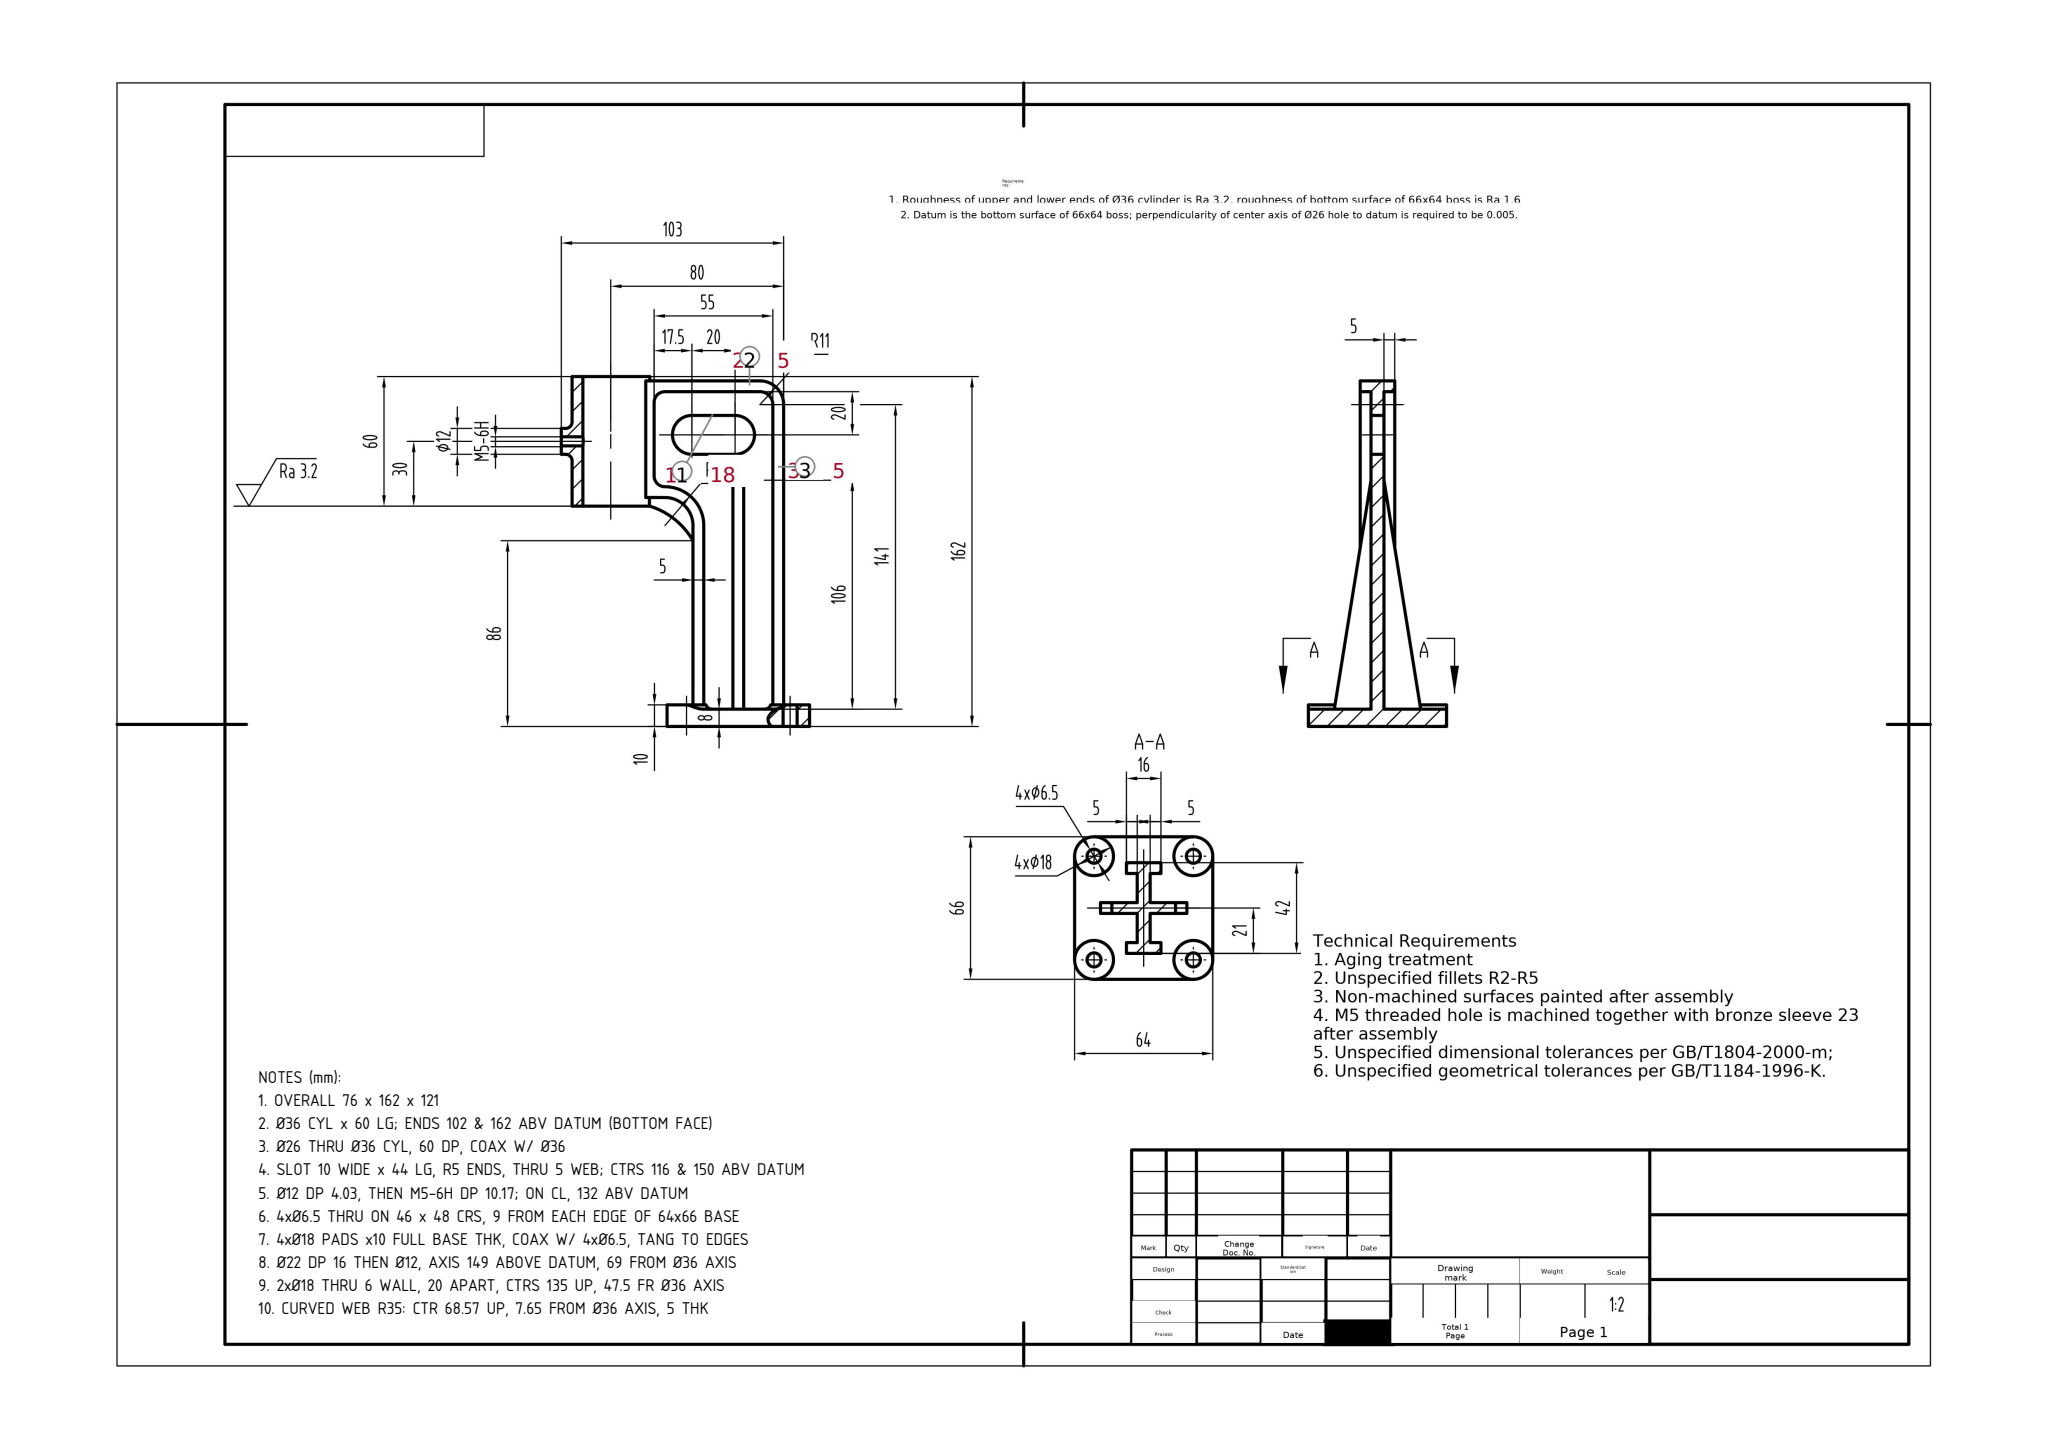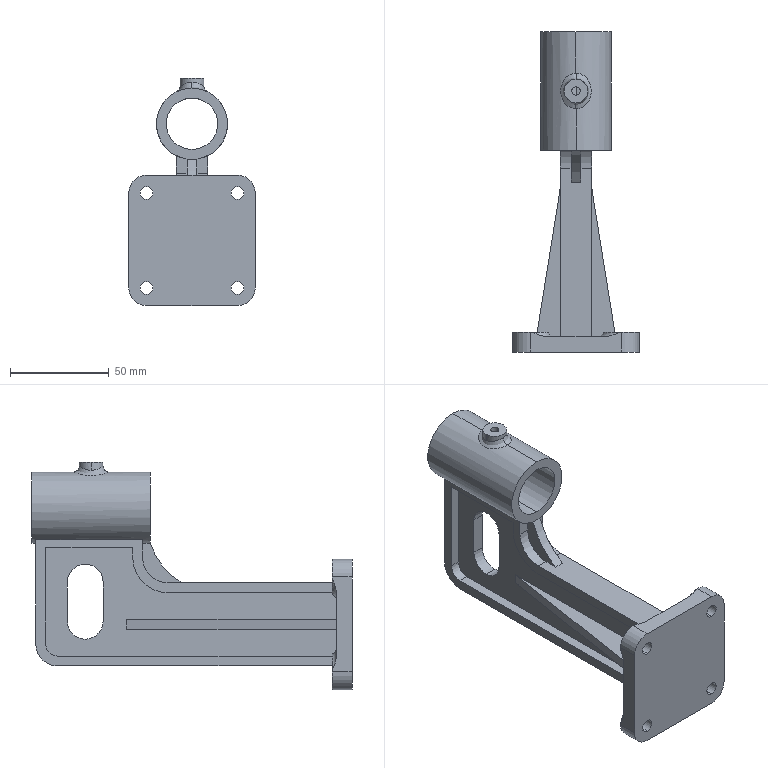Part | SolidWorks | mm | 1 solid | 83 faces | box 64 x 162 x 115 mm | volume 132433 mm3 | plane 41 | cylinder 33 | torus 7 | spline 2 | commonest cylinder face diameters 6.5 x8 18 x7 26 x4 12 x4 36 x4 4.2 x2 10 x2 22 x1
Drawing notes:
OVERALL 76 x 162 x 121 | from the solid: bbox_xyz 76.218 x 162.001 x 121.11
Ø36 CYL x 60 LG; ENDS 102 & 162 ABV DATUM (BOTTOM FACE) | from the solid: cyl dia 36, axis y, pos (x38.11,z98.11), len 60; y-planes 102 & 162
Ø26 THRU Ø36 CYL, 60 DP, COAX W/ Ø36 | from the solid: cyl dia 26, axis y, pos (x38.11,z98.11), len 60 = same as Ø36 boss
SLOT 10 WIDE x 44 LG, R5 ENDS, THRU 5 WEB; CTRS 116 & 150 ABV DATUM | from the solid: 2x cyl dia 10, axis x, at (y116,z73.11) & (y150,z73.11), len 5; web x35.61-40.61 = 5 thk
Ø12 DP 4.03, THEN M5-6H DP 10.17; ON CL, 132 ABV DATUM | from the solid: cyl dia 12 axis z len 4.03 and dia 4.2 tap drill axis z len 10.17 at (x38.11,y132)
4xØ6.5 THRU ON 46 x 48 CRS, 9 FROM EACH EDGE OF 64x66 BASE | from the solid: Ø6.5 y-axis holes at (x,z)=(15.11,15.11),(15.11,63.11),(61.11,15.11),(61.11,63.11); spacing 46 x 48; base faces x=6.11/70.11 (64) and z=6.11/72.11 (66) give 9 edge dist
4xØ18 PADS x10 FULL BASE THK, COAX W/ 4xØ6.5, TANG TO EDGES | from the solid: Ø18 y-axis cylinders L=10 at same 4 centres as Ø6.5; base plate y=0 to y=10; centres 9 from edges = R9 tangent
Ø22 DP 16 THEN Ø12, AXIS 149 ABOVE DATUM, 69 FROM Ø36 AXIS | from the solid: Ø22 x-axis cyl L=16 at (y,z)=(149,29.11); Ø12 x-axis L=5 same axis; Ø36 y-axis at z=98.11 -> 98.11-29.11=69
2xØ18 THRU 6 WALL, 20 APART, CTRS 135 UP, 47.5 FR Ø36 AXIS | from the solid: Ø18 x-axis cyls L=6 at (y,z)=(135,40.61) and (135,60.61); midpoint z=50.61; 98.11-50.61=47.5
CURVED WEB R35: CTR 68.57 UP, 7.65 FROM Ø36 AXIS, 5 THK | from the solid: Ø70 x-axis cyl L=5 at (y,z)=(68.57,90.46); R35; 98.11-90.46=7.65